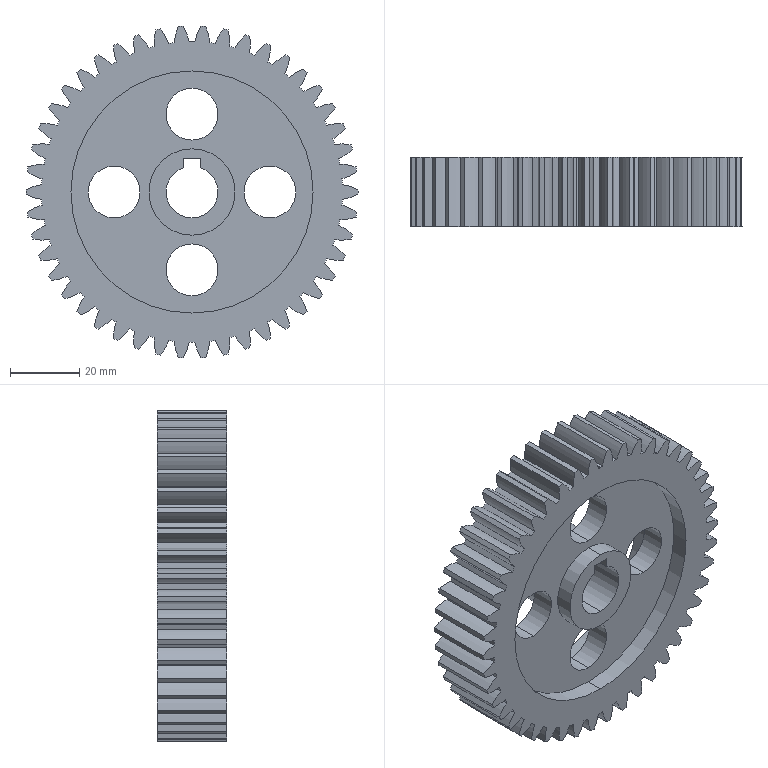Component | SolidWorks | 46-ToothGear-1 | 1 solid | 212 faces | volume 79442 mm3 | cylinder 111 | spline 92 | plane 9 | commonest cylinder face diameters 87 x47 96 x46 15 x10 25 x4 70 x4